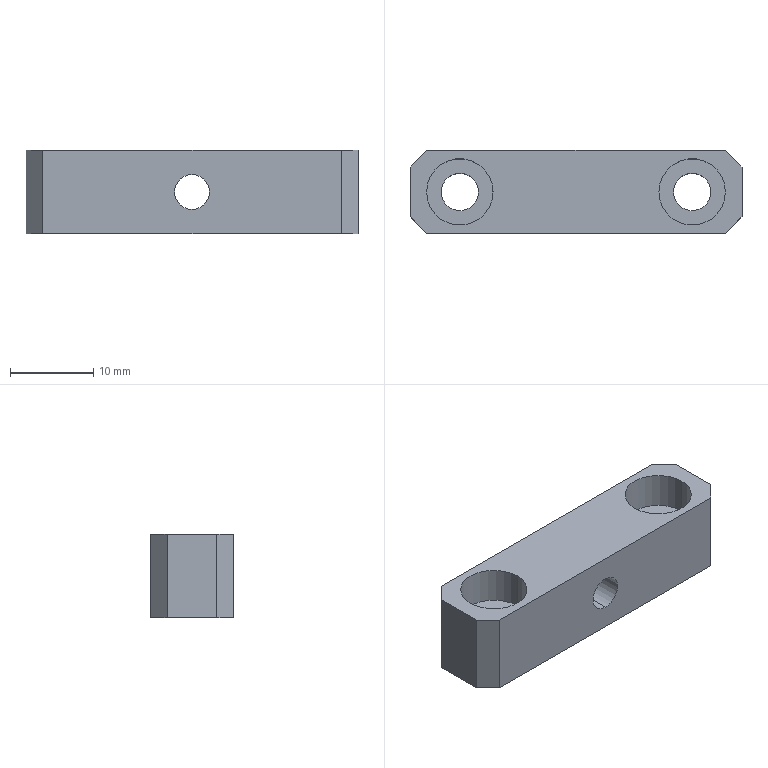Component | SolidWorks | DC-024-39-1 | 1 solid | 22 faces | box 40 x 10 x 10 mm | volume 3161 mm3 | plane 12 | cylinder 10 | commonest cylinder face diameters 8 x4 4.5 x4 4.2 x2
build123d program:
from build123d import *

# Parameters (mm, degrees)
SKETCH1_W                                       = 40
SKETCH1_H                                       = 10
BOSS_EXTRUDE1_DEPTH                             = 5
M4_HEX_SOCKET_HEAD_CAP_SCREW_CBORE1_D           = 4.5
M4_HEX_SOCKET_HEAD_CAP_SCREW_CBORE1_CBORE_D     = 8
M4_HEX_SOCKET_HEAD_CAP_SCREW_CBORE1_CBORE_DEPTH = 4.4
M5_TAPPED_HOLE1_D                               = 4.2
CHAMFER1_SIZE                                   = 2


with BuildPart() as part:
    # Sketch1 → Boss-Extrude1 (new, symmetric)
    with BuildSketch(Plane.XY):
        Rectangle(SKETCH1_W, SKETCH1_H)
    extrude(amount=BOSS_EXTRUDE1_DEPTH, both=True)

    # M4 Hex Socket Head Cap Screw CBORE1 (through all)
    with Locations(Plane.XY.offset(5)):
        with Locations((-14, 0), (14, 0)):
            CounterBoreHole(M4_HEX_SOCKET_HEAD_CAP_SCREW_CBORE1_D / 2, M4_HEX_SOCKET_HEAD_CAP_SCREW_CBORE1_CBORE_D / 2, M4_HEX_SOCKET_HEAD_CAP_SCREW_CBORE1_CBORE_DEPTH)

    # M5 Tapped Hole1 (through all)
    with Locations(Plane(origin=(0, -5, 0), x_dir=(-1, 0, 0), z_dir=(0, -1, 0))):
        with Locations((0, 0)):
            Hole(M5_TAPPED_HOLE1_D / 2)

    # Chamfer1
    chamfer1_edges = [part.edges().sort_by_distance(p)[0] for p in [
        (-20, 5, 0),
        (20, 5, 0),
        (20, -5, 0),
        (-20, -5, 0),
    ]]
    chamfer(chamfer1_edges, length=CHAMFER1_SIZE)


solid = part.part

# Placed as in the assembly
solid = solid.moved(Location((-25.633, 213.409, 18), (0, 0, 0)))
STEP:
#1=CARTESIAN_POINT('',(-1.009,8.599,0.7913));
#2=VERTEX_POINT('',#1);
#3=CARTESIAN_POINT('',(-1.009,8.599,0.626));
#4=VERTEX_POINT('',#3);
#5=CARTESIAN_POINT('',(-1.009,8.599,0.7087));
#6=DIRECTION('',(0.,-1.,0.));
#7=DIRECTION('',(0.,0.,-1.));
#8=AXIS2_PLACEMENT_3D('',#5,#6,#7);
#9=CIRCLE('',#8,0.08268);
#10=EDGE_CURVE('',#2,#4,#9,.T.);
#11=ORIENTED_EDGE('',*,*,#10,.F.);
#12=CARTESIAN_POINT('',(-1.009,8.205,0.7913));
#13=VERTEX_POINT('',#12);
#14=CARTESIAN_POINT('',(-1.009,8.205,0.7913));
#15=DIRECTION('',(0.,-1.,0.));
#16=VECTOR('',#15,39.37);
#17=LINE('',#14,#16);
#18=EDGE_CURVE('',#2,#13,#17,.T.);
#19=ORIENTED_EDGE('',*,*,#18,.T.);
#20=CARTESIAN_POINT('',(-1.009,8.205,0.626));
#21=VERTEX_POINT('',#20);
#22=CARTESIAN_POINT('',(-1.009,8.205,0.7087));
#23=DIRECTION('',(0.,-1.,0.));
#24=DIRECTION('',(0.,0.,-1.));
#25=AXIS2_PLACEMENT_3D('',#22,#23,#24);
#26=CIRCLE('',#25,0.08268);
#27=EDGE_CURVE('',#13,#21,#26,.T.);
#28=ORIENTED_EDGE('',*,*,#27,.T.);
#29=CARTESIAN_POINT('',(-1.009,8.205,0.626));
#30=DIRECTION('',(0.,-1.,0.));
#31=VECTOR('',#30,39.37);
#32=LINE('',#29,#31);
#33=EDGE_CURVE('',#4,#21,#32,.T.);
#34=ORIENTED_EDGE('',*,*,#33,.F.);
#35=EDGE_LOOP('',(#11,#19,#28,#34));
#36=FACE_OUTER_BOUND('',#35,.T.);
#37=CARTESIAN_POINT('',(-1.009,8.205,0.7087));
#38=DIRECTION('',(0.,-1.,0.));
#39=DIRECTION('',(0.,0.,-1.));
#40=AXIS2_PLACEMENT_3D('',#37,#38,#39);
#41=CYLINDRICAL_SURFACE('',#40,0.08268);
#42=ADVANCED_FACE('',(#36),#41,.F.);
#43=CARTESIAN_POINT('',(-1.718,8.402,0.7323));
#44=VERTEX_POINT('',#43);
#45=CARTESIAN_POINT('',(-1.403,8.402,0.7323));
#46=VERTEX_POINT('',#45);
#47=CARTESIAN_POINT('',(-1.56,8.402,0.7323));
#48=DIRECTION('',(0.,0.,1.));
#49=DIRECTION('',(1.,0.,0.));
#50=AXIS2_PLACEMENT_3D('',#47,#48,#49);
#51=CIRCLE('',#50,0.1575);
#52=EDGE_CURVE('',#44,#46,#51,.T.);
#53=ORIENTED_EDGE('',*,*,#52,.F.);
#54=CARTESIAN_POINT('',(-1.718,8.402,0.9055));
#55=VERTEX_POINT('',#54);
#56=CARTESIAN_POINT('',(-1.718,8.402,0.9055));
#57=DIRECTION('',(0.,0.,1.));
#58=VECTOR('',#57,39.37);
#59=LINE('',#56,#58);
#60=EDGE_CURVE('',#44,#55,#59,.T.);
#61=ORIENTED_EDGE('',*,*,#60,.T.);
#62=CARTESIAN_POINT('',(-1.403,8.402,0.9055));
#63=VERTEX_POINT('',#62);
#64=CARTESIAN_POINT('',(-1.56,8.402,0.9055));
#65=DIRECTION('',(0.,0.,1.));
#66=DIRECTION('',(1.,0.,0.));
#67=AXIS2_PLACEMENT_3D('',#64,#65,#66);
#68=CIRCLE('',#67,0.1575);
#69=EDGE_CURVE('',#55,#63,#68,.T.);
#70=ORIENTED_EDGE('',*,*,#69,.T.);
#71=CARTESIAN_POINT('',(-1.403,8.402,0.9055));
#72=DIRECTION('',(0.,0.,1.));
#73=VECTOR('',#72,39.37);
#74=LINE('',#71,#73);
#75=EDGE_CURVE('',#46,#63,#74,.T.);
#76=ORIENTED_EDGE('',*,*,#75,.F.);
#77=EDGE_LOOP('',(#53,#61,#70,#76));
#78=FACE_OUTER_BOUND('',#77,.T.);
#79=CARTESIAN_POINT('',(-1.56,8.402,0.9055));
#80=DIRECTION('',(0.,0.,1.));
#81=DIRECTION('',(1.,0.,0.));
#82=AXIS2_PLACEMENT_3D('',#79,#80,#81);
#83=CYLINDRICAL_SURFACE('',#82,0.1575);
#84=ADVANCED_FACE('',(#78),#83,.F.);
#85=CARTESIAN_POINT('',(-1.649,8.402,0.5118));
#86=VERTEX_POINT('',#85);
#87=CARTESIAN_POINT('',(-1.472,8.402,0.5118));
#88=VERTEX_POINT('',#87);
#89=CARTESIAN_POINT('',(-1.56,8.402,0.5118));
#90=DIRECTION('',(0.,0.,1.));
#91=DIRECTION('',(1.,0.,0.));
#92=AXIS2_PLACEMENT_3D('',#89,#90,#91);
#93=CIRCLE('',#92,0.08858);
#94=EDGE_CURVE('',#86,#88,#93,.T.);
#95=ORIENTED_EDGE('',*,*,#94,.F.);
#96=CARTESIAN_POINT('',(-1.649,8.402,0.7323));
#97=VERTEX_POINT('',#96);
#98=CARTESIAN_POINT('',(-1.649,8.402,0.9055));
#99=DIRECTION('',(0.,0.,1.));
#100=VECTOR('',#99,39.37);
#101=LINE('',#98,#100);
#102=EDGE_CURVE('',#86,#97,#101,.T.);
#103=ORIENTED_EDGE('',*,*,#102,.T.);
#104=CARTESIAN_POINT('',(-1.472,8.402,0.7323));
#105=VERTEX_POINT('',#104);
#106=CARTESIAN_POINT('',(-1.56,8.402,0.7323));
#107=DIRECTION('',(0.,0.,1.));
#108=DIRECTION('',(1.,0.,0.));
#109=AXIS2_PLACEMENT_3D('',#106,#107,#108);
#110=CIRCLE('',#109,0.08858);
#111=EDGE_CURVE('',#97,#105,#110,.T.);
#112=ORIENTED_EDGE('',*,*,#111,.T.);
#113=CARTESIAN_POINT('',(-1.472,8.402,0.9055));
#114=DIRECTION('',(0.,0.,1.));
#115=VECTOR('',#114,39.37);
#116=LINE('',#113,#115);
#117=EDGE_CURVE('',#88,#105,#116,.T.);
#118=ORIENTED_EDGE('',*,*,#117,.F.);
#119=EDGE_LOOP('',(#95,#103,#112,#118));
#120=FACE_OUTER_BOUND('',#119,.T.);
#121=CARTESIAN_POINT('',(-1.56,8.402,0.9055));
#122=DIRECTION('',(0.,0.,1.));
#123=DIRECTION('',(1.,0.,0.));
#124=AXIS2_PLACEMENT_3D('',#121,#122,#123);
#125=CYLINDRICAL_SURFACE('',#124,0.08858);
#126=ADVANCED_FACE('',(#120),#125,.F.);
#127=CARTESIAN_POINT('',(-0.6155,8.402,0.7323));
#128=VERTEX_POINT('',#127);
#129=CARTESIAN_POINT('',(-0.3005,8.402,0.7323));
#130=VERTEX_POINT('',#129);
#131=CARTESIAN_POINT('',(-0.458,8.402,0.7323));
#132=DIRECTION('',(0.,0.,1.));
#133=DIRECTION('',(1.,0.,0.));
#134=AXIS2_PLACEMENT_3D('',#131,#132,#133);
#135=CIRCLE('',#134,0.1575);
#136=EDGE_CURVE('',#128,#130,#135,.T.);
#137=ORIENTED_EDGE('',*,*,#136,.F.);
#138=CARTESIAN_POINT('',(-0.6155,8.402,0.9055));
#139=VERTEX_POINT('',#138);
#140=CARTESIAN_POINT('',(-0.6155,8.402,0.9055));
#141=DIRECTION('',(0.,0.,1.));
#142=VECTOR('',#141,39.37);
#143=LINE('',#140,#142);
#144=EDGE_CURVE('',#128,#139,#143,.T.);
#145=ORIENTED_EDGE('',*,*,#144,.T.);
#146=CARTESIAN_POINT('',(-0.3005,8.402,0.9055));
#147=VERTEX_POINT('',#146);
#148=CARTESIAN_POINT('',(-0.458,8.402,0.9055));
#149=DIRECTION('',(0.,0.,1.));
#150=DIRECTION('',(1.,0.,0.));
#151=AXIS2_PLACEMENT_3D('',#148,#149,#150);
#152=CIRCLE('',#151,0.1575);
#153=EDGE_CURVE('',#139,#147,#152,.T.);
#154=ORIENTED_EDGE('',*,*,#153,.T.);
#155=CARTESIAN_POINT('',(-0.3005,8.402,0.9055));
#156=DIRECTION('',(0.,0.,1.));
#157=VECTOR('',#156,39.37);
#158=LINE('',#155,#157);
#159=EDGE_CURVE('',#130,#147,#158,.T.);
#160=ORIENTED_EDGE('',*,*,#159,.F.);
#161=EDGE_LOOP('',(#137,#145,#154,#160));
#162=FACE_OUTER_BOUND('',#161,.T.);
#163=CARTESIAN_POINT('',(-0.458,8.402,0.9055));
#164=DIRECTION('',(0.,0.,1.));
#165=DIRECTION('',(1.,0.,0.));
#166=AXIS2_PLACEMENT_3D('',#163,#164,#165);
#167=CYLINDRICAL_SURFACE('',#166,0.1575);
#168=ADVANCED_FACE('',(#162),#167,.F.);
#169=CARTESIAN_POINT('',(-0.5466,8.402,0.5118));
#170=VERTEX_POINT('',#169);
#171=CARTESIAN_POINT('',(-0.3694,8.402,0.5118));
#172=VERTEX_POINT('',#171);
#173=CARTESIAN_POINT('',(-0.458,8.402,0.5118));
#174=DIRECTION('',(0.,0.,1.));
#175=DIRECTION('',(1.,0.,0.));
#176=AXIS2_PLACEMENT_3D('',#173,#174,#175);
#177=CIRCLE('',#176,0.08858);
#178=EDGE_CURVE('',#170,#172,#177,.T.);
#179=ORIENTED_EDGE('',*,*,#178,.F.);
#180=CARTESIAN_POINT('',(-0.5466,8.402,0.7323));
#181=VERTEX_POINT('',#180);
#182=CARTESIAN_POINT('',(-0.5466,8.402,0.9055));
#183=DIRECTION('',(0.,0.,1.));
#184=VECTOR('',#183,39.37);
#185=LINE('',#182,#184);
#186=EDGE_CURVE('',#170,#181,#185,.T.);
#187=ORIENTED_EDGE('',*,*,#186,.T.);
#188=CARTESIAN_POINT('',(-0.3694,8.402,0.7323));
#189=VERTEX_POINT('',#188);
#190=CARTESIAN_POINT('',(-0.458,8.402,0.7323));
#191=DIRECTION('',(0.,0.,1.));
#192=DIRECTION('',(1.,0.,0.));
#193=AXIS2_PLACEMENT_3D('',#190,#191,#192);
#194=CIRCLE('',#193,0.08858);
#195=EDGE_CURVE('',#181,#189,#194,.T.);
#196=ORIENTED_EDGE('',*,*,#195,.T.);
#197=CARTESIAN_POINT('',(-0.3694,8.402,0.9055));
#198=DIRECTION('',(0.,0.,1.));
#199=VECTOR('',#198,39.37);
#200=LINE('',#197,#199);
#201=EDGE_CURVE('',#172,#189,#200,.T.);
#202=ORIENTED_EDGE('',*,*,#201,.F.);
#203=EDGE_LOOP('',(#179,#187,#196,#202));
#204=FACE_OUTER_BOUND('',#203,.T.);
#205=CARTESIAN_POINT('',(-0.458,8.402,0.9055));
#206=DIRECTION('',(0.,0.,1.));
#207=DIRECTION('',(1.,0.,0.));
#208=AXIS2_PLACEMENT_3D('',#205,#206,#207);
#209=CYLINDRICAL_SURFACE('',#208,0.08858);
#210=ADVANCED_FACE('',(#204),#209,.F.);
#211=CARTESIAN_POINT('',(-1.797,8.52,0.9055));
#212=VERTEX_POINT('',#211);
#213=CARTESIAN_POINT('',(-1.797,8.284,0.9055));
#214=VERTEX_POINT('',#213);
#215=CARTESIAN_POINT('',(-1.797,8.205,0.9055));
#216=DIRECTION('',(0.,-1.,0.));
#217=VECTOR('',#216,39.37);
#218=LINE('',#215,#217);
#219=EDGE_CURVE('',#212,#214,#218,.T.);
#220=ORIENTED_EDGE('',*,*,#219,.F.);
#221=CARTESIAN_POINT('',(-1.797,8.52,0.5118));
#222=VERTEX_POINT('',#221);
#223=CARTESIAN_POINT('',(-1.797,8.52,0.9055));
#224=DIRECTION('',(0.,0.,-1.));
#225=VECTOR('',#224,39.37);
#226=LINE('',#223,#225);
#227=EDGE_CURVE('',#212,#222,#226,.T.);
#228=ORIENTED_EDGE('',*,*,#227,.T.);
#229=CARTESIAN_POINT('',(-1.797,8.284,0.5118));
#230=VERTEX_POINT('',#229);
#231=CARTESIAN_POINT('',(-1.797,8.205,0.5118));
#232=DIRECTION('',(0.,-1.,0.));
#233=VECTOR('',#232,39.37);
#234=LINE('',#231,#233);
#235=EDGE_CURVE('',#222,#230,#234,.T.);
#236=ORIENTED_EDGE('',*,*,#235,.T.);
#237=CARTESIAN_POINT('',(-1.797,8.284,0.9055));
#238=DIRECTION('',(0.,0.,1.));
#239=VECTOR('',#238,39.37);
#240=LINE('',#237,#239);
#241=EDGE_CURVE('',#230,#214,#240,.T.);
#242=ORIENTED_EDGE('',*,*,#241,.T.);
#243=EDGE_LOOP('',(#220,#228,#236,#242));
#244=FACE_OUTER_BOUND('',#243,.T.);
#245=CARTESIAN_POINT('',(-1.797,8.205,0.9055));
#246=DIRECTION('',(1.,0.,0.));
#247=DIRECTION('',(0.,0.,-1.));
#248=AXIS2_PLACEMENT_3D('',#245,#246,#247);
#249=PLANE('',#248);
#250=ADVANCED_FACE('',(#244),#249,.F.);
#251=CARTESIAN_POINT('',(-1.009,8.205,0.7087));
#252=DIRECTION('',(0.,-1.,0.));
#253=DIRECTION('',(0.,0.,-1.));
#254=AXIS2_PLACEMENT_3D('',#251,#252,#253);
#255=CIRCLE('',#254,0.08268);
#256=EDGE_CURVE('',#21,#13,#255,.T.);
#257=ORIENTED_EDGE('',*,*,#256,.F.);
#258=ORIENTED_EDGE('',*,*,#27,.F.);
#259=EDGE_LOOP('',(#257,#258));
#260=FACE_BOUND('',#259,.T.);
#261=CARTESIAN_POINT('',(-1.718,8.205,0.5118));
#262=VERTEX_POINT('',#261);
#263=CARTESIAN_POINT('',(-0.3005,8.205,0.5118));
#264=VERTEX_POINT('',#263);
#265=CARTESIAN_POINT('',(-0.2218,8.205,0.5118));
#266=DIRECTION('',(1.,0.,0.));
#267=VECTOR('',#266,39.37);
#268=LINE('',#265,#267);
#269=EDGE_CURVE('',#262,#264,#268,.T.);
#270=ORIENTED_EDGE('',*,*,#269,.T.);
#271=CARTESIAN_POINT('',(-0.3005,8.205,0.9055));
#272=VERTEX_POINT('',#271);
#273=CARTESIAN_POINT('',(-0.3005,8.205,0.9055));
#274=DIRECTION('',(0.,0.,1.));
#275=VECTOR('',#274,39.37);
#276=LINE('',#273,#275);
#277=EDGE_CURVE('',#264,#272,#276,.T.);
#278=ORIENTED_EDGE('',*,*,#277,.T.);
#279=CARTESIAN_POINT('',(-1.718,8.205,0.9055));
#280=VERTEX_POINT('',#279);
#281=CARTESIAN_POINT('',(-0.2218,8.205,0.9055));
#282=DIRECTION('',(1.,0.,0.));
#283=VECTOR('',#282,39.37);
#284=LINE('',#281,#283);
#285=EDGE_CURVE('',#280,#272,#284,.T.);
#286=ORIENTED_EDGE('',*,*,#285,.F.);
#287=CARTESIAN_POINT('',(-1.718,8.205,0.9055));
#288=DIRECTION('',(0.,0.,-1.));
#289=VECTOR('',#288,39.37);
#290=LINE('',#287,#289);
#291=EDGE_CURVE('',#280,#262,#290,.T.);
#292=ORIENTED_EDGE('',*,*,#291,.T.);
#293=EDGE_LOOP('',(#270,#278,#286,#292));
#294=FACE_OUTER_BOUND('',#293,.T.);
#295=CARTESIAN_POINT('',(-0.2218,8.205,0.9055));
#296=DIRECTION('',(0.,1.,0.));
#297=DIRECTION('',(0.,0.,1.));
#298=AXIS2_PLACEMENT_3D('',#295,#296,#297);
#299=PLANE('',#298);
#300=ADVANCED_FACE('',(#260,#294),#299,.F.);
#301=CARTESIAN_POINT('',(-0.2218,8.284,0.5118));
#302=VERTEX_POINT('',#301);
#303=CARTESIAN_POINT('',(-0.2218,8.52,0.5118));
#304=VERTEX_POINT('',#303);
#305=CARTESIAN_POINT('',(-0.2218,8.205,0.5118));
#306=DIRECTION('',(0.,1.,0.));
#307=VECTOR('',#306,39.37);
#308=LINE('',#305,#307);
#309=EDGE_CURVE('',#302,#304,#308,.T.);
#310=ORIENTED_EDGE('',*,*,#309,.T.);
#311=CARTESIAN_POINT('',(-0.2218,8.52,0.9055));
#312=VERTEX_POINT('',#311);
#313=CARTESIAN_POINT('',(-0.2218,8.52,0.9055));
#314=DIRECTION('',(0.,0.,1.));
#315=VECTOR('',#314,39.37);
#316=LINE('',#313,#315);
#317=EDGE_CURVE('',#304,#312,#316,.T.);
#318=ORIENTED_EDGE('',*,*,#317,.T.);
#319=CARTESIAN_POINT('',(-0.2218,8.284,0.9055));
#320=VERTEX_POINT('',#319);
#321=CARTESIAN_POINT('',(-0.2218,8.205,0.9055));
#322=DIRECTION('',(0.,1.,0.));
#323=VECTOR('',#322,39.37);
#324=LINE('',#321,#323);
#325=EDGE_CURVE('',#320,#312,#324,.T.);
#326=ORIENTED_EDGE('',*,*,#325,.F.);
#327=CARTESIAN_POINT('',(-0.2218,8.284,0.9055));
#328=DIRECTION('',(0.,0.,-1.));
#329=VECTOR('',#328,39.37);
#330=LINE('',#327,#329);
#331=EDGE_CURVE('',#320,#302,#330,.T.);
#332=ORIENTED_EDGE('',*,*,#331,.T.);
#333=EDGE_LOOP('',(#310,#318,#326,#332));
#334=FACE_OUTER_BOUND('',#333,.T.);
#335=CARTESIAN_POINT('',(-0.2218,8.205,0.9055));
#336=DIRECTION('',(-1.,0.,0.));
#337=DIRECTION('',(0.,0.,1.));
#338=AXIS2_PLACEMENT_3D('',#335,#336,#337);
#339=PLANE('',#338);
#340=ADVANCED_FACE('',(#334),#339,.F.);
#341=CARTESIAN_POINT('',(-1.009,8.599,0.7087));
#342=DIRECTION('',(0.,-1.,0.));
#343=DIRECTION('',(0.,0.,-1.));
#344=AXIS2_PLACEMENT_3D('',#341,#342,#343);
#345=CIRCLE('',#344,0.08268);
#346=EDGE_CURVE('',#4,#2,#345,.T.);
#347=ORIENTED_EDGE('',*,*,#346,.T.);
#348=ORIENTED_EDGE('',*,*,#10,.T.);
#349=EDGE_LOOP('',(#347,#348));
#350=FACE_BOUND('',#349,.T.);
#351=CARTESIAN_POINT('',(-0.3005,8.599,0.9055));
#352=VERTEX_POINT('',#351);
#353=CARTESIAN_POINT('',(-1.718,8.599,0.9055));
#354=VERTEX_POINT('',#353);
#355=CARTESIAN_POINT('',(-0.2218,8.599,0.9055));
#356=DIRECTION('',(-1.,0.,0.));
#357=VECTOR('',#356,39.37);
#358=LINE('',#355,#357);
#359=EDGE_CURVE('',#352,#354,#358,.T.);
#360=ORIENTED_EDGE('',*,*,#359,.F.);
#361=CARTESIAN_POINT('',(-0.3005,8.599,0.5118));
#362=VERTEX_POINT('',#361);
#363=CARTESIAN_POINT('',(-0.3005,8.599,0.9055));
#364=DIRECTION('',(0.,0.,-1.));
#365=VECTOR('',#364,39.37);
#366=LINE('',#363,#365);
#367=EDGE_CURVE('',#352,#362,#366,.T.);
#368=ORIENTED_EDGE('',*,*,#367,.T.);
#369=CARTESIAN_POINT('',(-1.718,8.599,0.5118));
#370=VERTEX_POINT('',#369);
#371=CARTESIAN_POINT('',(-0.2218,8.599,0.5118));
#372=DIRECTION('',(-1.,0.,0.));
#373=VECTOR('',#372,39.37);
#374=LINE('',#371,#373);
#375=EDGE_CURVE('',#362,#370,#374,.T.);
#376=ORIENTED_EDGE('',*,*,#375,.T.);
#377=CARTESIAN_POINT('',(-1.718,8.599,0.9055));
#378=DIRECTION('',(0.,0.,1.));
#379=VECTOR('',#378,39.37);
#380=LINE('',#377,#379);
#381=EDGE_CURVE('',#370,#354,#380,.T.);
#382=ORIENTED_EDGE('',*,*,#381,.T.);
#383=EDGE_LOOP('',(#360,#368,#376,#382));
#384=FACE_OUTER_BOUND('',#383,.T.);
#385=CARTESIAN_POINT('',(-0.2218,8.599,0.9055));
#386=DIRECTION('',(0.,-1.,0.));
#387=DIRECTION('',(0.,0.,-1.));
#388=AXIS2_PLACEMENT_3D('',#385,#386,#387);
#389=PLANE('',#388);
#390=ADVANCED_FACE('',(#350,#384),#389,.F.);
#391=CARTESIAN_POINT('',(-1.56,8.402,0.9055));
#392=DIRECTION('',(0.,0.,1.));
#393=DIRECTION('',(1.,0.,0.));
#394=AXIS2_PLACEMENT_3D('',#391,#392,#393);
#395=CIRCLE('',#394,0.1575);
#396=EDGE_CURVE('',#63,#55,#395,.T.);
#397=ORIENTED_EDGE('',*,*,#396,.F.);
#398=ORIENTED_EDGE('',*,*,#69,.F.);
#399=EDGE_LOOP('',(#397,#398));
#400=FACE_BOUND('',#399,.T.);
#401=CARTESIAN_POINT('',(-0.458,8.402,0.9055));
#402=DIRECTION('',(0.,0.,1.));
#403=DIRECTION('',(1.,0.,0.));
#404=AXIS2_PLACEMENT_3D('',#401,#402,#403);
#405=CIRCLE('',#404,0.1575);
#406=EDGE_CURVE('',#147,#139,#405,.T.);
#407=ORIENTED_EDGE('',*,*,#406,.F.);
#408=ORIENTED_EDGE('',*,*,#153,.F.);
#409=EDGE_LOOP('',(#407,#408));
#410=FACE_BOUND('',#409,.T.);
#411=ORIENTED_EDGE('',*,*,#325,.T.);
#412=CARTESIAN_POINT('',(-0.5564,8.855,0.9055));
#413=DIRECTION('',(-0.7071,0.7071,0.));
#414=VECTOR('',#413,39.37);
#415=LINE('',#412,#414);
#416=EDGE_CURVE('',#312,#352,#415,.T.);
#417=ORIENTED_EDGE('',*,*,#416,.T.);
#418=ORIENTED_EDGE('',*,*,#359,.T.);
#419=CARTESIAN_POINT('',(-1.462,8.855,0.9055));
#420=DIRECTION('',(-0.7071,-0.7071,0.));
#421=VECTOR('',#420,39.37);
#422=LINE('',#419,#421);
#423=EDGE_CURVE('',#354,#212,#422,.T.);
#424=ORIENTED_EDGE('',*,*,#423,.T.);
#425=ORIENTED_EDGE('',*,*,#219,.T.);
#426=CARTESIAN_POINT('',(-1.462,7.949,0.9055));
#427=DIRECTION('',(0.7071,-0.7071,0.));
#428=VECTOR('',#427,39.37);
#429=LINE('',#426,#428);
#430=EDGE_CURVE('',#214,#280,#429,.T.);
#431=ORIENTED_EDGE('',*,*,#430,.T.);
#432=ORIENTED_EDGE('',*,*,#285,.T.);
#433=CARTESIAN_POINT('',(-0.5564,7.949,0.9055));
#434=DIRECTION('',(0.7071,0.7071,0.));
#435=VECTOR('',#434,39.37);
#436=LINE('',#433,#435);
#437=EDGE_CURVE('',#272,#320,#436,.T.);
#438=ORIENTED_EDGE('',*,*,#437,.T.);
#439=EDGE_LOOP('',(#411,#417,#418,#424,#425,#431,#432,#438));
#440=FACE_OUTER_BOUND('',#439,.T.);
#441=CARTESIAN_POINT('',(-1.009,8.402,0.9055));
#442=DIRECTION('',(0.,0.,1.));
#443=DIRECTION('',(1.,0.,0.));
#444=AXIS2_PLACEMENT_3D('',#441,#442,#443);
#445=PLANE('',#444);
#446=ADVANCED_FACE('',(#400,#410,#440),#445,.T.);
#447=CARTESIAN_POINT('',(-1.56,8.402,0.5118));
#448=DIRECTION('',(0.,0.,1.));
#449=DIRECTION('',(1.,0.,0.));
#450=AXIS2_PLACEMENT_3D('',#447,#448,#449);
#451=CIRCLE('',#450,0.08858);
#452=EDGE_CURVE('',#88,#86,#451,.T.);
#453=ORIENTED_EDGE('',*,*,#452,.T.);
#454=ORIENTED_EDGE('',*,*,#94,.T.);
#455=EDGE_LOOP('',(#453,#454));
#456=FACE_BOUND('',#455,.T.);
#457=CARTESIAN_POINT('',(-0.458,8.402,0.5118));
#458=DIRECTION('',(0.,0.,1.));
#459=DIRECTION('',(1.,0.,0.));
#460=AXIS2_PLACEMENT_3D('',#457,#458,#459);
#461=CIRCLE('',#460,0.08858);
#462=EDGE_CURVE('',#172,#170,#461,.T.);
#463=ORIENTED_EDGE('',*,*,#462,.T.);
#464=ORIENTED_EDGE('',*,*,#178,.T.);
#465=EDGE_LOOP('',(#463,#464));
#466=FACE_BOUND('',#465,.T.);
#467=ORIENTED_EDGE('',*,*,#375,.F.);
#468=CARTESIAN_POINT('',(-0.3005,8.599,0.5118));
#469=DIRECTION('',(0.7071,-0.7071,0.));
#470=VECTOR('',#469,39.37);
#471=LINE('',#468,#470);
#472=EDGE_CURVE('',#362,#304,#471,.T.);
#473=ORIENTED_EDGE('',*,*,#472,.T.);
#474=ORIENTED_EDGE('',*,*,#309,.F.);
#475=CARTESIAN_POINT('',(-0.2218,8.284,0.5118));
#476=DIRECTION('',(-0.7071,-0.7071,0.));
#477=VECTOR('',#476,39.37);
#478=LINE('',#475,#477);
#479=EDGE_CURVE('',#302,#264,#478,.T.);
#480=ORIENTED_EDGE('',*,*,#479,.T.);
#481=ORIENTED_EDGE('',*,*,#269,.F.);
#482=CARTESIAN_POINT('',(-1.718,8.205,0.5118));
#483=DIRECTION('',(-0.7071,0.7071,0.));
#484=VECTOR('',#483,39.37);
#485=LINE('',#482,#484);
#486=EDGE_CURVE('',#262,#230,#485,.T.);
#487=ORIENTED_EDGE('',*,*,#486,.T.);
#488=ORIENTED_EDGE('',*,*,#235,.F.);
#489=CARTESIAN_POINT('',(-1.797,8.52,0.5118));
#490=DIRECTION('',(0.7071,0.7071,0.));
#491=VECTOR('',#490,39.37);
#492=LINE('',#489,#491);
#493=EDGE_CURVE('',#222,#370,#492,.T.);
#494=ORIENTED_EDGE('',*,*,#493,.T.);
#495=EDGE_LOOP('',(#467,#473,#474,#480,#481,#487,#488,#494));
#496=FACE_OUTER_BOUND('',#495,.T.);
#497=CARTESIAN_POINT('',(-1.009,8.402,0.5118));
#498=DIRECTION('',(0.,0.,1.));
#499=DIRECTION('',(1.,0.,0.));
#500=AXIS2_PLACEMENT_3D('',#497,#498,#499);
#501=PLANE('',#500);
#502=ADVANCED_FACE('',(#456,#466,#496),#501,.F.);
#503=ORIENTED_EDGE('',*,*,#186,.F.);
#504=ORIENTED_EDGE('',*,*,#462,.F.);
#505=ORIENTED_EDGE('',*,*,#201,.T.);
#506=CARTESIAN_POINT('',(-0.458,8.402,0.7323));
#507=DIRECTION('',(0.,0.,1.));
#508=DIRECTION('',(1.,0.,0.));
#509=AXIS2_PLACEMENT_3D('',#506,#507,#508);
#510=CIRCLE('',#509,0.08858);
#511=EDGE_CURVE('',#189,#181,#510,.T.);
#512=ORIENTED_EDGE('',*,*,#511,.T.);
#513=EDGE_LOOP('',(#503,#504,#505,#512));
#514=FACE_OUTER_BOUND('',#513,.T.);
#515=CARTESIAN_POINT('',(-0.458,8.402,0.9055));
#516=DIRECTION('',(0.,0.,1.));
#517=DIRECTION('',(1.,0.,0.));
#518=AXIS2_PLACEMENT_3D('',#515,#516,#517);
#519=CYLINDRICAL_SURFACE('',#518,0.08858);
#520=ADVANCED_FACE('',(#514),#519,.F.);
#521=ORIENTED_EDGE('',*,*,#511,.F.);
#522=ORIENTED_EDGE('',*,*,#195,.F.);
#523=EDGE_LOOP('',(#521,#522));
#524=FACE_BOUND('',#523,.T.);
#525=CARTESIAN_POINT('',(-0.458,8.402,0.7323));
#526=DIRECTION('',(0.,0.,1.));
#527=DIRECTION('',(1.,0.,0.));
#528=AXIS2_PLACEMENT_3D('',#525,#526,#527);
#529=CIRCLE('',#528,0.1575);
#530=EDGE_CURVE('',#130,#128,#529,.T.);
#531=ORIENTED_EDGE('',*,*,#530,.T.);
#532=ORIENTED_EDGE('',*,*,#136,.T.);
#533=EDGE_LOOP('',(#531,#532));
#534=FACE_OUTER_BOUND('',#533,.T.);
#535=CARTESIAN_POINT('',(-0.3694,8.402,0.7323));
#536=DIRECTION('',(0.,0.,-1.));
#537=DIRECTION('',(-1.,0.,0.));
#538=AXIS2_PLACEMENT_3D('',#535,#536,#537);
#539=PLANE('',#538);
#540=ADVANCED_FACE('',(#524,#534),#539,.F.);
#541=ORIENTED_EDGE('',*,*,#144,.F.);
#542=ORIENTED_EDGE('',*,*,#530,.F.);
#543=ORIENTED_EDGE('',*,*,#159,.T.);
#544=ORIENTED_EDGE('',*,*,#406,.T.);
#545=EDGE_LOOP('',(#541,#542,#543,#544));
#546=FACE_OUTER_BOUND('',#545,.T.);
#547=CARTESIAN_POINT('',(-0.458,8.402,0.9055));
#548=DIRECTION('',(0.,0.,1.));
#549=DIRECTION('',(1.,0.,0.));
#550=AXIS2_PLACEMENT_3D('',#547,#548,#549);
#551=CYLINDRICAL_SURFACE('',#550,0.1575);
#552=ADVANCED_FACE('',(#546),#551,.F.);
#553=ORIENTED_EDGE('',*,*,#102,.F.);
#554=ORIENTED_EDGE('',*,*,#452,.F.);
#555=ORIENTED_EDGE('',*,*,#117,.T.);
#556=CARTESIAN_POINT('',(-1.56,8.402,0.7323));
#557=DIRECTION('',(0.,0.,1.));
#558=DIRECTION('',(1.,0.,0.));
#559=AXIS2_PLACEMENT_3D('',#556,#557,#558);
#560=CIRCLE('',#559,0.08858);
#561=EDGE_CURVE('',#105,#97,#560,.T.);
#562=ORIENTED_EDGE('',*,*,#561,.T.);
#563=EDGE_LOOP('',(#553,#554,#555,#562));
#564=FACE_OUTER_BOUND('',#563,.T.);
#565=CARTESIAN_POINT('',(-1.56,8.402,0.9055));
#566=DIRECTION('',(0.,0.,1.));
#567=DIRECTION('',(1.,0.,0.));
#568=AXIS2_PLACEMENT_3D('',#565,#566,#567);
#569=CYLINDRICAL_SURFACE('',#568,0.08858);
#570=ADVANCED_FACE('',(#564),#569,.F.);
#571=ORIENTED_EDGE('',*,*,#561,.F.);
#572=ORIENTED_EDGE('',*,*,#111,.F.);
#573=EDGE_LOOP('',(#571,#572));
#574=FACE_BOUND('',#573,.T.);
#575=CARTESIAN_POINT('',(-1.56,8.402,0.7323));
#576=DIRECTION('',(0.,0.,1.));
#577=DIRECTION('',(1.,0.,0.));
#578=AXIS2_PLACEMENT_3D('',#575,#576,#577);
#579=CIRCLE('',#578,0.1575);
#580=EDGE_CURVE('',#46,#44,#579,.T.);
#581=ORIENTED_EDGE('',*,*,#580,.T.);
#582=ORIENTED_EDGE('',*,*,#52,.T.);
#583=EDGE_LOOP('',(#581,#582));
#584=FACE_OUTER_BOUND('',#583,.T.);
#585=CARTESIAN_POINT('',(-1.472,8.402,0.7323));
#586=DIRECTION('',(0.,0.,-1.));
#587=DIRECTION('',(-1.,0.,0.));
#588=AXIS2_PLACEMENT_3D('',#585,#586,#587);
#589=PLANE('',#588);
#590=ADVANCED_FACE('',(#574,#584),#589,.F.);
#591=ORIENTED_EDGE('',*,*,#60,.F.);
#592=ORIENTED_EDGE('',*,*,#580,.F.);
#593=ORIENTED_EDGE('',*,*,#75,.T.);
#594=ORIENTED_EDGE('',*,*,#396,.T.);
#595=EDGE_LOOP('',(#591,#592,#593,#594));
#596=FACE_OUTER_BOUND('',#595,.T.);
#597=CARTESIAN_POINT('',(-1.56,8.402,0.9055));
#598=DIRECTION('',(0.,0.,1.));
#599=DIRECTION('',(1.,0.,0.));
#600=AXIS2_PLACEMENT_3D('',#597,#598,#599);
#601=CYLINDRICAL_SURFACE('',#600,0.1575);
#602=ADVANCED_FACE('',(#596),#601,.F.);
#603=ORIENTED_EDGE('',*,*,#18,.F.);
#604=ORIENTED_EDGE('',*,*,#346,.F.);
#605=ORIENTED_EDGE('',*,*,#33,.T.);
#606=ORIENTED_EDGE('',*,*,#256,.T.);
#607=EDGE_LOOP('',(#603,#604,#605,#606));
#608=FACE_OUTER_BOUND('',#607,.T.);
#609=CARTESIAN_POINT('',(-1.009,8.205,0.7087));
#610=DIRECTION('',(0.,-1.,0.));
#611=DIRECTION('',(0.,0.,-1.));
#612=AXIS2_PLACEMENT_3D('',#609,#610,#611);
#613=CYLINDRICAL_SURFACE('',#612,0.08268);
#614=ADVANCED_FACE('',(#608),#613,.F.);
#615=ORIENTED_EDGE('',*,*,#416,.F.);
#616=ORIENTED_EDGE('',*,*,#317,.F.);
#617=ORIENTED_EDGE('',*,*,#472,.F.);
#618=ORIENTED_EDGE('',*,*,#367,.F.);
#619=EDGE_LOOP('',(#615,#616,#617,#618));
#620=FACE_OUTER_BOUND('',#619,.T.);
#621=CARTESIAN_POINT('',(-0.3005,8.599,0.9055));
#622=DIRECTION('',(-0.7071,-0.7071,0.));
#623=DIRECTION('',(0.,0.,-1.));
#624=AXIS2_PLACEMENT_3D('',#621,#622,#623);
#625=PLANE('',#624);
#626=ADVANCED_FACE('',(#620),#625,.F.);
#627=ORIENTED_EDGE('',*,*,#437,.F.);
#628=ORIENTED_EDGE('',*,*,#277,.F.);
#629=ORIENTED_EDGE('',*,*,#479,.F.);
#630=ORIENTED_EDGE('',*,*,#331,.F.);
#631=EDGE_LOOP('',(#627,#628,#629,#630));
#632=FACE_OUTER_BOUND('',#631,.T.);
#633=CARTESIAN_POINT('',(-0.2218,8.284,0.9055));
#634=DIRECTION('',(-0.7071,0.7071,0.));
#635=DIRECTION('',(0.,0.,-1.));
#636=AXIS2_PLACEMENT_3D('',#633,#634,#635);
#637=PLANE('',#636);
#638=ADVANCED_FACE('',(#632),#637,.F.);
#639=ORIENTED_EDGE('',*,*,#423,.F.);
#640=ORIENTED_EDGE('',*,*,#381,.F.);
#641=ORIENTED_EDGE('',*,*,#493,.F.);
#642=ORIENTED_EDGE('',*,*,#227,.F.);
#643=EDGE_LOOP('',(#639,#640,#641,#642));
#644=FACE_OUTER_BOUND('',#643,.T.);
#645=CARTESIAN_POINT('',(-1.797,8.52,0.9055));
#646=DIRECTION('',(0.7071,-0.7071,0.));
#647=DIRECTION('',(0.,0.,-1.));
#648=AXIS2_PLACEMENT_3D('',#645,#646,#647);
#649=PLANE('',#648);
#650=ADVANCED_FACE('',(#644),#649,.F.);
#651=ORIENTED_EDGE('',*,*,#430,.F.);
#652=ORIENTED_EDGE('',*,*,#241,.F.);
#653=ORIENTED_EDGE('',*,*,#486,.F.);
#654=ORIENTED_EDGE('',*,*,#291,.F.);
#655=EDGE_LOOP('',(#651,#652,#653,#654));
#656=FACE_OUTER_BOUND('',#655,.T.);
#657=CARTESIAN_POINT('',(-1.718,8.205,0.9055));
#658=DIRECTION('',(0.7071,0.7071,0.));
#659=DIRECTION('',(0.,0.,-1.));
#660=AXIS2_PLACEMENT_3D('',#657,#658,#659);
#661=PLANE('',#660);
#662=ADVANCED_FACE('',(#656),#661,.F.);
#663=CLOSED_SHELL('',(#42,#84,#126,#168,#210,#250,#300,#340,#390,#446,#502,#520,#540,#552,#570,#590,#602,#614,#626,#638,#650,#662));
#664=MANIFOLD_SOLID_BREP('',#663);
#665=CARTESIAN_POINT('',(0.,0.,0.));
#666=DIRECTION('',(0.,0.,1.));
#667=DIRECTION('',(1.,0.,0.));
#668=AXIS2_PLACEMENT_3D('',#665,#666,#667);
#669=(LENGTH_UNIT()NAMED_UNIT(*)SI_UNIT($,.METRE.));
#670=LENGTH_MEASURE_WITH_UNIT(LENGTH_MEASURE(0.0254),#669);
#671=DIMENSIONAL_EXPONENTS(1.,0.,0.,0.,0.,0.,0.);
#672=(CONVERSION_BASED_UNIT('',#670)LENGTH_UNIT()NAMED_UNIT(#671));
#673=UNCERTAINTY_MEASURE_WITH_UNIT(LENGTH_MEASURE(0.00001),#672,'','');
#674=(NAMED_UNIT(*)PLANE_ANGLE_UNIT()SI_UNIT($,.RADIAN.));
#675=(NAMED_UNIT(*)SI_UNIT($,.STERADIAN.)SOLID_ANGLE_UNIT());
#676=(GEOMETRIC_REPRESENTATION_CONTEXT(3)GLOBAL_UNCERTAINTY_ASSIGNED_CONTEXT((#673))GLOBAL_UNIT_ASSIGNED_CONTEXT((#672,#674,#675))REPRESENTATION_CONTEXT('',''));
#677=ADVANCED_BREP_SHAPE_REPRESENTATION('',(#664,#668),#676);
#678=COLOUR_RGB('',0.7922,0.8196,0.9333);
#679=FILL_AREA_STYLE_COLOUR('',#678);
#680=FILL_AREA_STYLE('',(#679));
#681=SURFACE_STYLE_FILL_AREA(#680);
#682=SURFACE_SIDE_STYLE('',(#681));
#683=SURFACE_STYLE_USAGE(.BOTH.,#682);
#684=PRESENTATION_STYLE_ASSIGNMENT((#683));
#685=STYLED_ITEM('',(#684),#664);
#686=(LENGTH_UNIT()NAMED_UNIT(*)SI_UNIT($,.METRE.));
#687=LENGTH_MEASURE_WITH_UNIT(LENGTH_MEASURE(0.0254),#686);
#688=DIMENSIONAL_EXPONENTS(1.,0.,0.,0.,0.,0.,0.);
#689=(CONVERSION_BASED_UNIT('',#687)LENGTH_UNIT()NAMED_UNIT(#688));
#690=UNCERTAINTY_MEASURE_WITH_UNIT(LENGTH_MEASURE(0.00001),#689,'','');
#691=(NAMED_UNIT(*)PLANE_ANGLE_UNIT()SI_UNIT($,.RADIAN.));
#692=(NAMED_UNIT(*)SI_UNIT($,.STERADIAN.)SOLID_ANGLE_UNIT());
#693=(GEOMETRIC_REPRESENTATION_CONTEXT(3)GLOBAL_UNCERTAINTY_ASSIGNED_CONTEXT((#690))GLOBAL_UNIT_ASSIGNED_CONTEXT((#689,#691,#692))REPRESENTATION_CONTEXT('',''));
#694=MECHANICAL_DESIGN_GEOMETRIC_PRESENTATION_REPRESENTATION('',(#685),#693);
#695=PRESENTATION_LAYER_ASSIGNMENT('','',(#685));